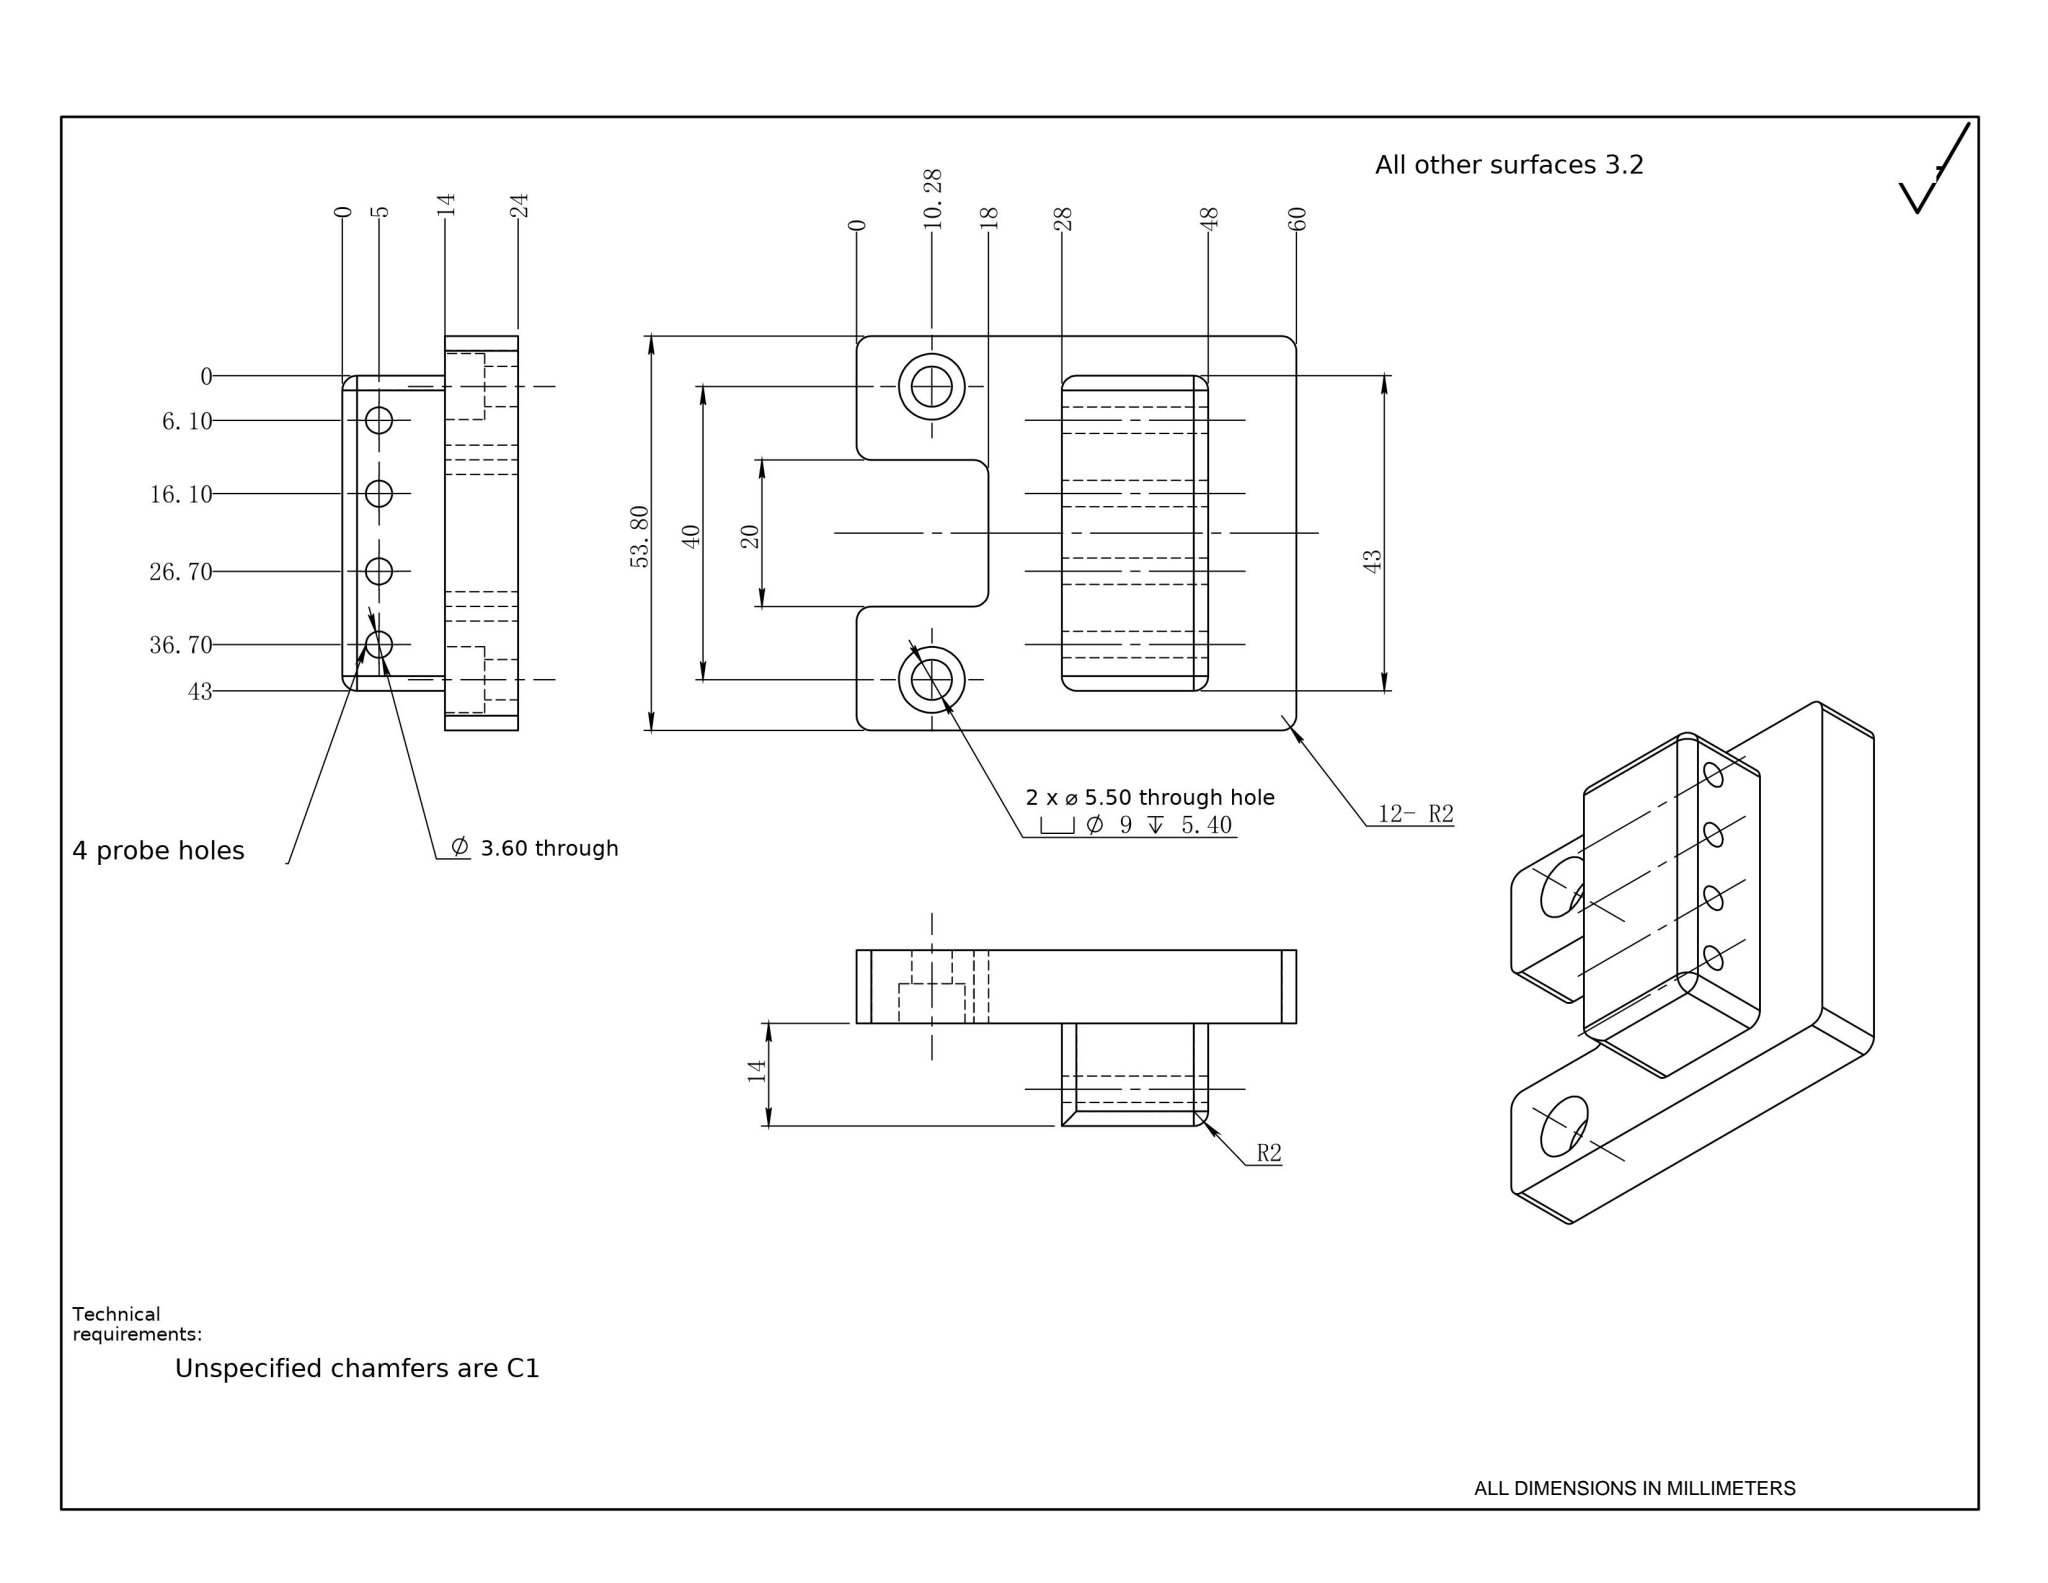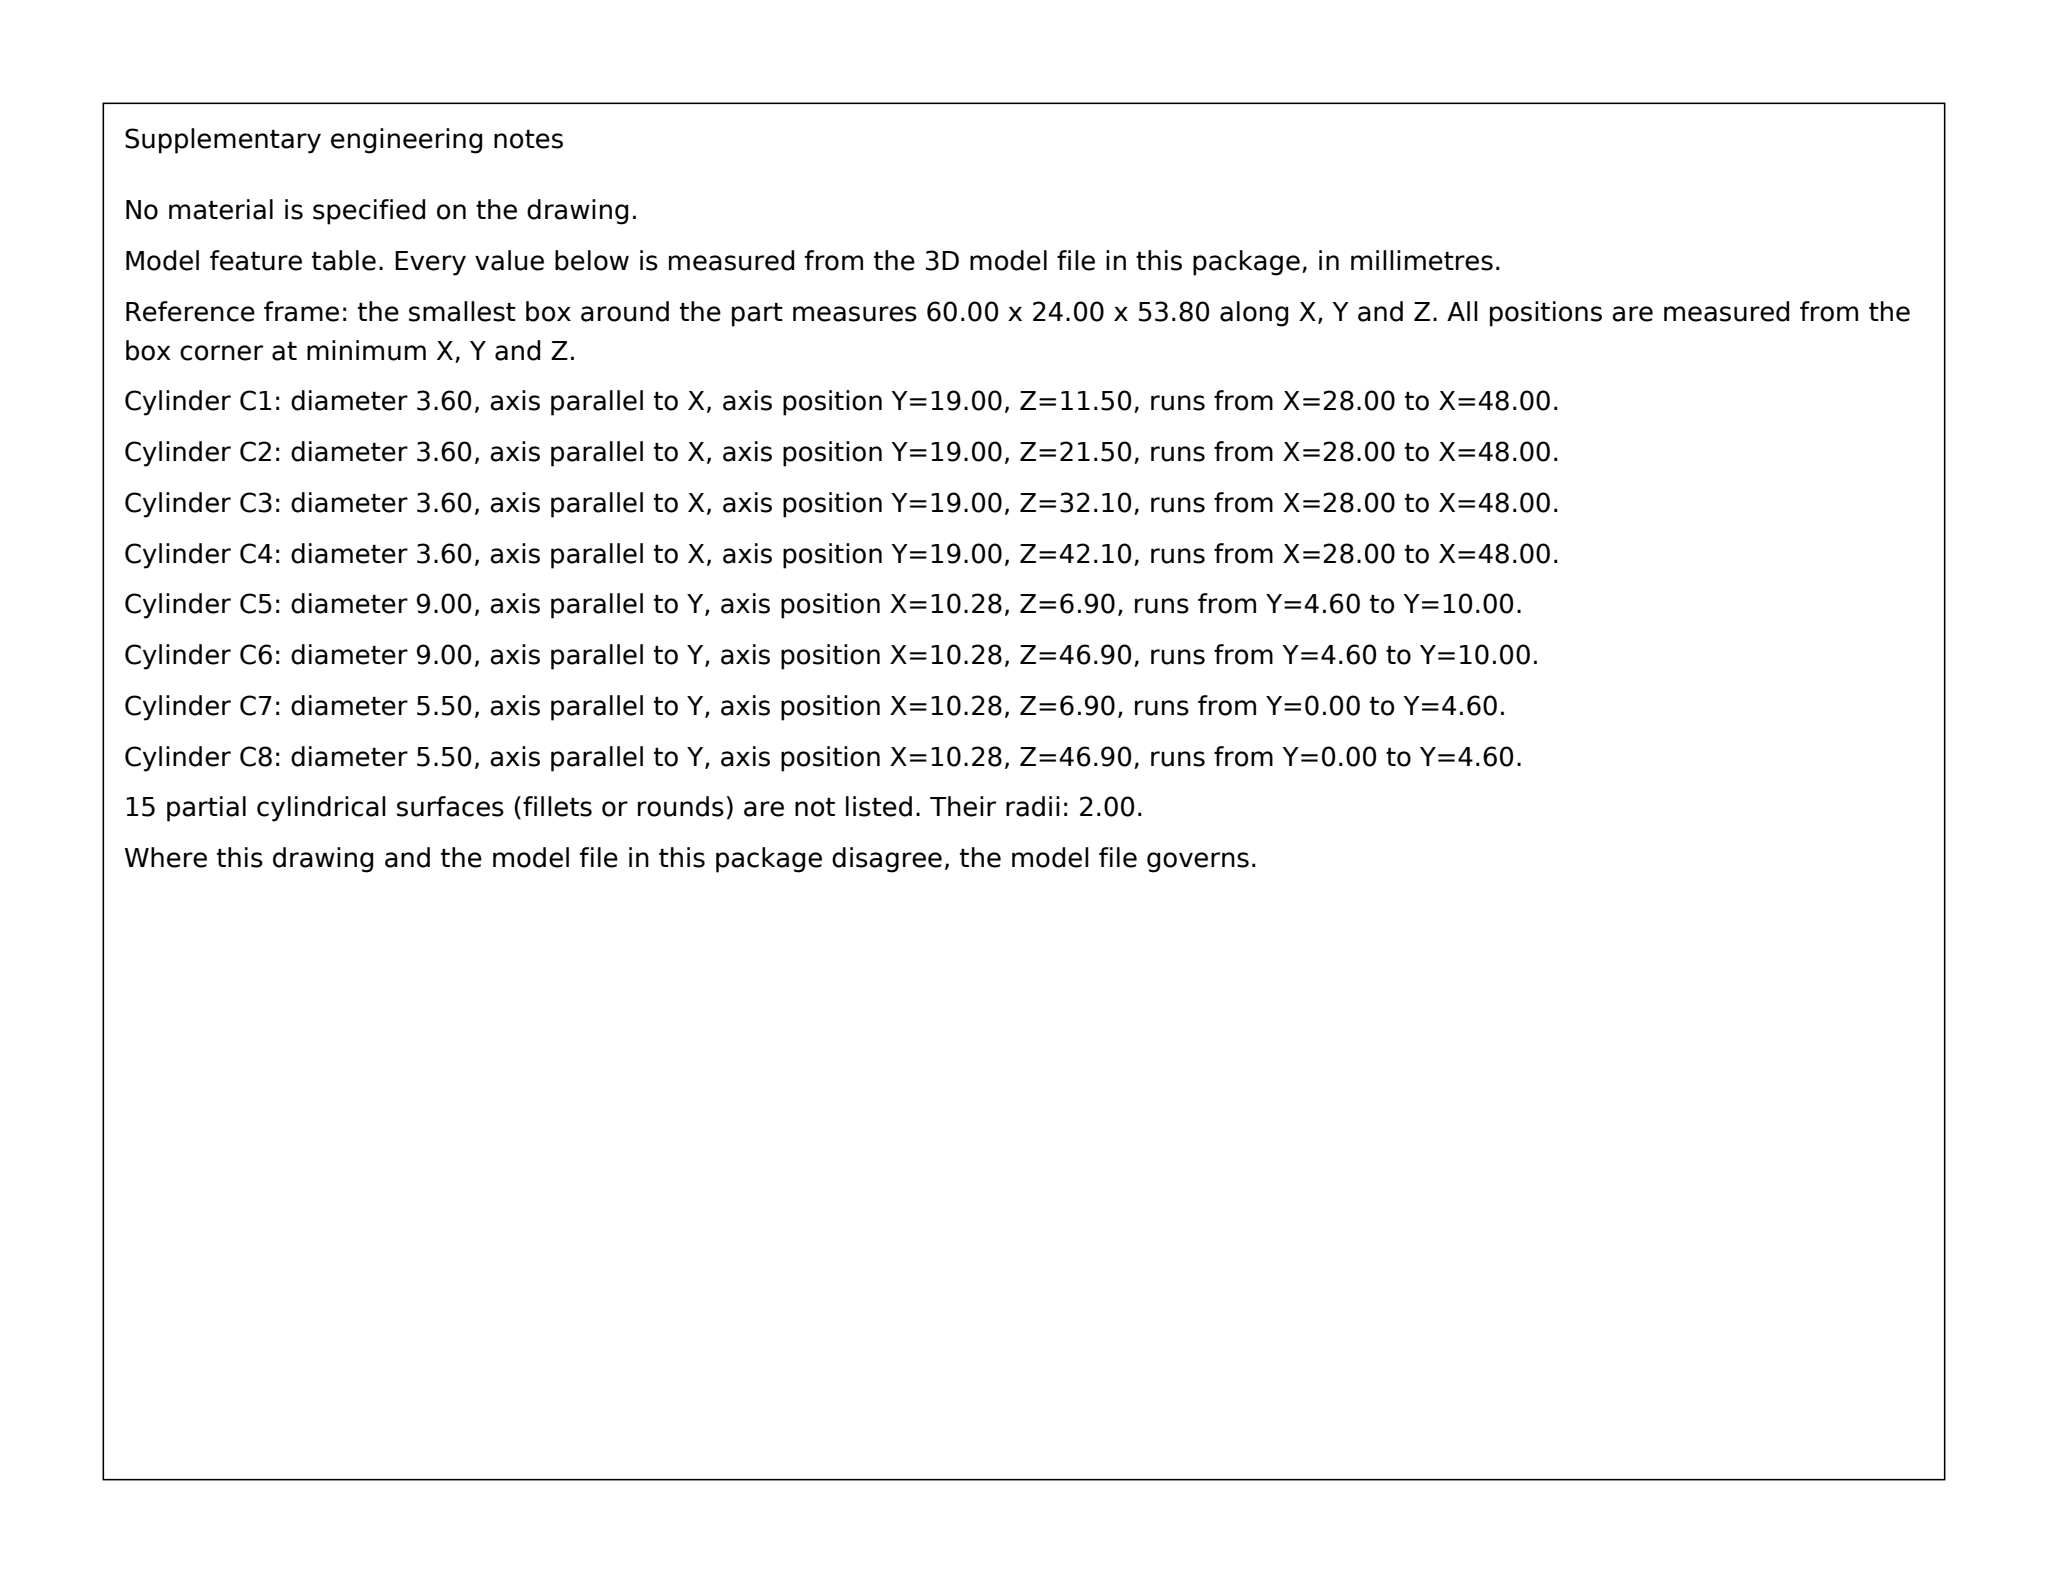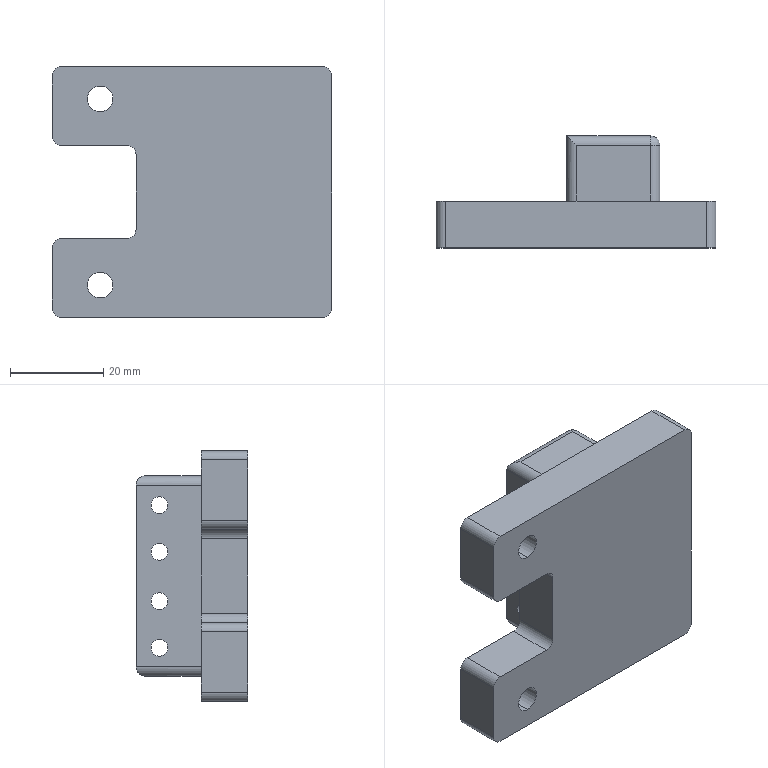Part | SolidWorks | mm | 1 solid | 50 faces | box 60 x 24 x 53.8 mm | volume 38851 mm3 | cylinder 31 | plane 17 | sphere 2 | commonest cylinder face diameters 4 x15 3.6 x8 9 x4 5.5 x4
build123d program:
from build123d import *

# Parameters (mm, degrees)
SKETCH1_W                                       = 60
SKETCH1_H                                       = 53.8
BOSS_EXTRUDE1_DEPTH                             = 24
SKETCH2_W                                       = 28
SKETCH2_H                                       = 14
CUT_EXTRUDE1_DEPTH                              = 60
M5_HEX_SOCKET_HEAD_CAP_SCREW_CBORE1_D           = 5.5
M5_HEX_SOCKET_HEAD_CAP_SCREW_CBORE1_CBORE_D     = 9
M5_HEX_SOCKET_HEAD_CAP_SCREW_CBORE1_CBORE_DEPTH = 5.4
SKETCH6_W                                       = 18
SKETCH6_H                                       = 20
CUT_EXTRUDE3_DEPTH                              = 10
SKETCH10_W                                      = 32
SKETCH10_H                                      = 5.4
CUT_EXTRUDE4_DEPTH                              = 14
SKETCH13_W                                      = 12
SKETCH13_H                                      = 43
CUT_EXTRUDE6_DEPTH                              = 14
SKETCH5_R                                       = 1.8
CUT_EXTRUDE2_DEPTH                              = 61.03
FILLET5_R                                       = 2


with BuildPart() as part:
    # Sketch1 → Boss-Extrude1 (new body)
    with BuildSketch(Plane(origin=(0, 0, 0), x_dir=(1, 0, 0), z_dir=(0, 1, 0))):
        Rectangle(SKETCH1_W, SKETCH1_H)
    extrude(amount=BOSS_EXTRUDE1_DEPTH)

    # Sketch2 → Cut-Extrude1 (cut)
    with BuildSketch(Plane.XY.offset(26.9)):
        with Locations((-16, 17)):
            Rectangle(SKETCH2_W, SKETCH2_H)
    extrude(amount=-CUT_EXTRUDE1_DEPTH, mode=Mode.SUBTRACT)

    # M5 Hex Socket Head Cap Screw CBORE1 (through all)
    with Locations(Plane(origin=(0, 10, 0), x_dir=(1, 0, 0), z_dir=(0, 1, 0))):
        with Locations((-19.721, 20), (-19.721, -20)):
            CounterBoreHole(M5_HEX_SOCKET_HEAD_CAP_SCREW_CBORE1_D / 2, M5_HEX_SOCKET_HEAD_CAP_SCREW_CBORE1_CBORE_D / 2, M5_HEX_SOCKET_HEAD_CAP_SCREW_CBORE1_CBORE_DEPTH)

    # Sketch6 → Cut-Extrude3 (cut)
    with BuildSketch(Plane(origin=(0, 10, 0), x_dir=(1, 0, 0), z_dir=(0, 1, 0))):
        with Locations((-21, 0)):
            Rectangle(SKETCH6_W, SKETCH6_H)
    extrude(amount=-CUT_EXTRUDE3_DEPTH, mode=Mode.SUBTRACT)

    # Sketch10 → Cut-Extrude4 (cut)
    with BuildSketch(Plane(origin=(0, 24, 0), x_dir=(1, 0, 0), z_dir=(0, 1, 0))):
        with Locations((14, 24.2)):
            Rectangle(SKETCH10_W, SKETCH10_H)
        with Locations((14, -24.2)):
            Rectangle(SKETCH10_W, SKETCH10_H)
    extrude(amount=-CUT_EXTRUDE4_DEPTH, mode=Mode.SUBTRACT)

    # Sketch13 → Cut-Extrude6 (cut)
    with BuildSketch(Plane(origin=(0, 24, 0), x_dir=(1, 0, 0), z_dir=(0, 1, 0))):
        with Locations((24, 0)):
            Rectangle(SKETCH13_W, SKETCH13_H)
    extrude(amount=-CUT_EXTRUDE6_DEPTH, mode=Mode.SUBTRACT)

    # Sketch5 → Cut-Extrude2 (cut, through all)
    with BuildSketch(Plane(origin=(18, 0, 0), x_dir=(0, 0, -1), z_dir=(1, 0, 0))):
        with Locations((15.4, 19)):
            Circle(SKETCH5_R)
        with Locations((5.4, 19)):
            Circle(SKETCH5_R)
        with Locations((-5.2, 19)):
            Circle(SKETCH5_R)
        with Locations((-15.2, 19)):
            Circle(SKETCH5_R)
    extrude(amount=-CUT_EXTRUDE2_DEPTH, mode=Mode.SUBTRACT)

    # Fillet5
    fillet5_edges = [part.edges().sort_by_distance(p)[0] for p in [
        (-30, 5, 26.9),
        (-30, 5, -26.9),
        (-30, 5, 10),
        (-30, 5, -10),
        (-12, 5, -10),
        (-12, 5, 10),
        (30, 5, 26.9),
        (30, 5, -26.9),
        (-2, 17, -21.5),
        (8, 24, -21.5),
        (-2, 17, 21.5),
        (8, 24, 21.5),
        (18, 17, 21.5),
        (18, 17, -21.5),
        (18, 24, 0),
    ]]
    fillet(fillet5_edges, radius=FILLET5_R)


solid = part.part